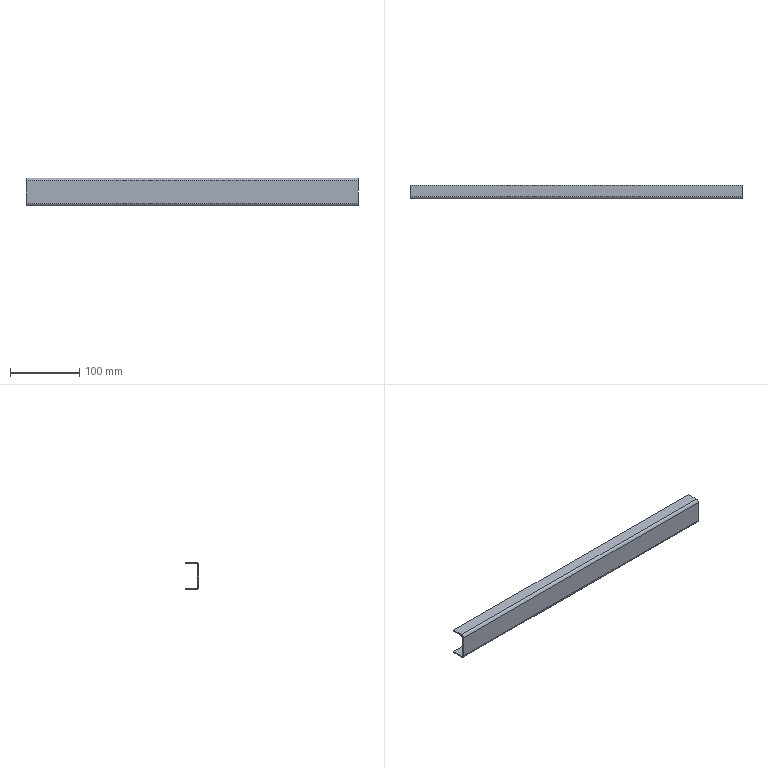Component | SolidWorks | ElectricalCabinetDoorAssembly-1_ElectricalCabinetDoorStiffener-1 | 1 solid | 22 faces | box 480 x 20 x 40 mm | volume 70488 mm3 | plane 18 | cylinder 4 | commonest cylinder face diameters 8 x2 4 x2 | material Plain Carbon Steel
STEP:
#1=COLOUR_RGB('',0.7922,0.8196,0.9333);
#2=FILL_AREA_STYLE_COLOUR('',#1);
#3=FILL_AREA_STYLE('',(#2));
#4=SURFACE_STYLE_FILL_AREA(#3);
#5=SURFACE_SIDE_STYLE('',(#4));
#6=SURFACE_STYLE_USAGE(.BOTH.,#5);
#7=PRESENTATION_STYLE_ASSIGNMENT((#6));
#8=CARTESIAN_POINT('',(96.921,48.88,54.212));
#9=VERTEX_POINT('',#8);
#10=CARTESIAN_POINT('',(96.921,48.959,54.212));
#11=VERTEX_POINT('',#10);
#12=CARTESIAN_POINT('',(96.921,48.88,54.212));
#13=DIRECTION('',(0.,1.,-0.));
#14=VECTOR('',#13,39.37);
#15=LINE('',#12,#14);
#16=EDGE_CURVE('',#9,#11,#15,.T.);
#17=ORIENTED_EDGE('',*,*,#16,.F.);
#18=CARTESIAN_POINT('',(96.921,49.037,54.054));
#19=VERTEX_POINT('',#18);
#20=CARTESIAN_POINT('',(96.921,49.037,54.212));
#21=DIRECTION('',(-1.,0.,0.));
#22=DIRECTION('',(0.,0.,1.));
#23=AXIS2_PLACEMENT_3D('',#20,#21,#22);
#24=CIRCLE('',#23,0.1575);
#25=EDGE_CURVE('',#19,#9,#24,.T.);
#26=ORIENTED_EDGE('',*,*,#25,.F.);
#27=CARTESIAN_POINT('',(96.921,49.037,54.133));
#28=VERTEX_POINT('',#27);
#29=CARTESIAN_POINT('',(96.921,49.037,54.133));
#30=DIRECTION('',(-0.,-0.,-1.));
#31=VECTOR('',#30,39.37);
#32=LINE('',#29,#31);
#33=EDGE_CURVE('',#28,#19,#32,.T.);
#34=ORIENTED_EDGE('',*,*,#33,.F.);
#35=CARTESIAN_POINT('',(96.921,49.037,54.212));
#36=DIRECTION('',(-1.,0.,0.));
#37=DIRECTION('',(0.,0.,1.));
#38=AXIS2_PLACEMENT_3D('',#35,#36,#37);
#39=CIRCLE('',#38,0.07874);
#40=EDGE_CURVE('',#28,#11,#39,.T.);
#41=ORIENTED_EDGE('',*,*,#40,.T.);
#42=EDGE_LOOP('',(#17,#26,#34,#41));
#43=FACE_OUTER_BOUND('',#42,.T.);
#44=CARTESIAN_POINT('',(96.921,48.88,54.212));
#45=DIRECTION('',(1.,-0.,-0.));
#46=DIRECTION('',(0.,0.,1.));
#47=AXIS2_PLACEMENT_3D('',#44,#45,#46);
#48=PLANE('',#47);
#49=ADVANCED_FACE('',(#43),#48,.T.);
#50=CARTESIAN_POINT('',(96.921,48.88,55.472));
#51=VERTEX_POINT('',#50);
#52=CARTESIAN_POINT('',(96.921,48.88,54.054));
#53=DIRECTION('',(0.,0.,1.));
#54=VECTOR('',#53,39.37);
#55=LINE('',#52,#54);
#56=EDGE_CURVE('',#9,#51,#55,.T.);
#57=ORIENTED_EDGE('',*,*,#56,.F.);
#58=ORIENTED_EDGE('',*,*,#16,.T.);
#59=CARTESIAN_POINT('',(96.921,48.959,55.472));
#60=VERTEX_POINT('',#59);
#61=CARTESIAN_POINT('',(96.921,48.959,54.054));
#62=DIRECTION('',(0.,0.,1.));
#63=VECTOR('',#62,39.37);
#64=LINE('',#61,#63);
#65=EDGE_CURVE('',#11,#60,#64,.T.);
#66=ORIENTED_EDGE('',*,*,#65,.T.);
#67=CARTESIAN_POINT('',(96.921,48.959,55.472));
#68=DIRECTION('',(-0.,-1.,0.));
#69=VECTOR('',#68,39.37);
#70=LINE('',#67,#69);
#71=EDGE_CURVE('',#60,#51,#70,.T.);
#72=ORIENTED_EDGE('',*,*,#71,.T.);
#73=EDGE_LOOP('',(#57,#58,#66,#72));
#74=FACE_OUTER_BOUND('',#73,.T.);
#75=CARTESIAN_POINT('',(96.921,49.037,54.133));
#76=DIRECTION('',(1.,-0.,-0.));
#77=DIRECTION('',(0.,0.,1.));
#78=AXIS2_PLACEMENT_3D('',#75,#76,#77);
#79=PLANE('',#78);
#80=ADVANCED_FACE('',(#74),#79,.T.);
#81=CARTESIAN_POINT('',(78.023,49.037,54.054));
#82=VERTEX_POINT('',#81);
#83=CARTESIAN_POINT('',(78.023,49.037,54.133));
#84=VERTEX_POINT('',#83);
#85=CARTESIAN_POINT('',(78.023,49.037,54.054));
#86=DIRECTION('',(0.,0.,1.));
#87=VECTOR('',#86,39.37);
#88=LINE('',#85,#87);
#89=EDGE_CURVE('',#82,#84,#88,.T.);
#90=ORIENTED_EDGE('',*,*,#89,.F.);
#91=CARTESIAN_POINT('',(78.023,48.88,54.212));
#92=VERTEX_POINT('',#91);
#93=CARTESIAN_POINT('',(78.023,49.037,54.212));
#94=DIRECTION('',(-1.,0.,0.));
#95=DIRECTION('',(0.,0.,1.));
#96=AXIS2_PLACEMENT_3D('',#93,#94,#95);
#97=CIRCLE('',#96,0.1575);
#98=EDGE_CURVE('',#82,#92,#97,.T.);
#99=ORIENTED_EDGE('',*,*,#98,.T.);
#100=CARTESIAN_POINT('',(78.023,48.959,54.212));
#101=VERTEX_POINT('',#100);
#102=CARTESIAN_POINT('',(78.023,48.959,54.212));
#103=DIRECTION('',(-0.,-1.,0.));
#104=VECTOR('',#103,39.37);
#105=LINE('',#102,#104);
#106=EDGE_CURVE('',#101,#92,#105,.T.);
#107=ORIENTED_EDGE('',*,*,#106,.F.);
#108=CARTESIAN_POINT('',(78.023,49.037,54.212));
#109=DIRECTION('',(-1.,0.,0.));
#110=DIRECTION('',(0.,0.,1.));
#111=AXIS2_PLACEMENT_3D('',#108,#109,#110);
#112=CIRCLE('',#111,0.07874);
#113=EDGE_CURVE('',#84,#101,#112,.T.);
#114=ORIENTED_EDGE('',*,*,#113,.F.);
#115=EDGE_LOOP('',(#90,#99,#107,#114));
#116=FACE_OUTER_BOUND('',#115,.T.);
#117=CARTESIAN_POINT('',(78.023,49.037,54.054));
#118=DIRECTION('',(-1.,0.,0.));
#119=DIRECTION('',(-0.,-0.,-1.));
#120=AXIS2_PLACEMENT_3D('',#117,#118,#119);
#121=PLANE('',#120);
#122=ADVANCED_FACE('',(#116),#121,.T.);
#123=CARTESIAN_POINT('',(78.023,49.667,54.054));
#124=VERTEX_POINT('',#123);
#125=CARTESIAN_POINT('',(78.023,49.667,54.054));
#126=DIRECTION('',(-0.,-1.,0.));
#127=VECTOR('',#126,39.37);
#128=LINE('',#125,#127);
#129=EDGE_CURVE('',#124,#82,#128,.T.);
#130=ORIENTED_EDGE('',*,*,#129,.T.);
#131=ORIENTED_EDGE('',*,*,#89,.T.);
#132=CARTESIAN_POINT('',(78.023,49.667,54.133));
#133=VERTEX_POINT('',#132);
#134=CARTESIAN_POINT('',(78.023,49.667,54.133));
#135=DIRECTION('',(-0.,-1.,0.));
#136=VECTOR('',#135,39.37);
#137=LINE('',#134,#136);
#138=EDGE_CURVE('',#133,#84,#137,.T.);
#139=ORIENTED_EDGE('',*,*,#138,.F.);
#140=CARTESIAN_POINT('',(78.023,49.667,54.133));
#141=DIRECTION('',(-0.,-0.,-1.));
#142=VECTOR('',#141,39.37);
#143=LINE('',#140,#142);
#144=EDGE_CURVE('',#133,#124,#143,.T.);
#145=ORIENTED_EDGE('',*,*,#144,.T.);
#146=EDGE_LOOP('',(#130,#131,#139,#145));
#147=FACE_OUTER_BOUND('',#146,.T.);
#148=CARTESIAN_POINT('',(78.023,48.959,54.212));
#149=DIRECTION('',(-1.,0.,0.));
#150=DIRECTION('',(-0.,-0.,-1.));
#151=AXIS2_PLACEMENT_3D('',#148,#149,#150);
#152=PLANE('',#151);
#153=ADVANCED_FACE('',(#147),#152,.T.);
#154=CARTESIAN_POINT('',(96.921,49.037,55.629));
#155=VERTEX_POINT('',#154);
#156=CARTESIAN_POINT('',(96.921,49.037,55.55));
#157=VERTEX_POINT('',#156);
#158=CARTESIAN_POINT('',(96.921,49.037,55.629));
#159=DIRECTION('',(-0.,-0.,-1.));
#160=VECTOR('',#159,39.37);
#161=LINE('',#158,#160);
#162=EDGE_CURVE('',#155,#157,#161,.T.);
#163=ORIENTED_EDGE('',*,*,#162,.F.);
#164=CARTESIAN_POINT('',(96.921,49.037,55.472));
#165=DIRECTION('',(-1.,0.,0.));
#166=DIRECTION('',(0.,0.,1.));
#167=AXIS2_PLACEMENT_3D('',#164,#165,#166);
#168=CIRCLE('',#167,0.1575);
#169=EDGE_CURVE('',#51,#155,#168,.T.);
#170=ORIENTED_EDGE('',*,*,#169,.F.);
#171=ORIENTED_EDGE('',*,*,#71,.F.);
#172=CARTESIAN_POINT('',(96.921,49.037,55.472));
#173=DIRECTION('',(-1.,0.,0.));
#174=DIRECTION('',(0.,0.,1.));
#175=AXIS2_PLACEMENT_3D('',#172,#173,#174);
#176=CIRCLE('',#175,0.07874);
#177=EDGE_CURVE('',#60,#157,#176,.T.);
#178=ORIENTED_EDGE('',*,*,#177,.T.);
#179=EDGE_LOOP('',(#163,#170,#171,#178));
#180=FACE_OUTER_BOUND('',#179,.T.);
#181=CARTESIAN_POINT('',(96.921,49.037,55.629));
#182=DIRECTION('',(1.,-0.,-0.));
#183=DIRECTION('',(0.,0.,1.));
#184=AXIS2_PLACEMENT_3D('',#181,#182,#183);
#185=PLANE('',#184);
#186=ADVANCED_FACE('',(#180),#185,.T.);
#187=CARTESIAN_POINT('',(96.921,49.667,55.629));
#188=VERTEX_POINT('',#187);
#189=CARTESIAN_POINT('',(96.921,48.88,55.629));
#190=DIRECTION('',(0.,1.,-0.));
#191=VECTOR('',#190,39.37);
#192=LINE('',#189,#191);
#193=EDGE_CURVE('',#155,#188,#192,.T.);
#194=ORIENTED_EDGE('',*,*,#193,.F.);
#195=ORIENTED_EDGE('',*,*,#162,.T.);
#196=CARTESIAN_POINT('',(96.921,49.667,55.55));
#197=VERTEX_POINT('',#196);
#198=CARTESIAN_POINT('',(96.921,48.88,55.55));
#199=DIRECTION('',(0.,1.,-0.));
#200=VECTOR('',#199,39.37);
#201=LINE('',#198,#200);
#202=EDGE_CURVE('',#157,#197,#201,.T.);
#203=ORIENTED_EDGE('',*,*,#202,.T.);
#204=CARTESIAN_POINT('',(96.921,49.667,55.629));
#205=DIRECTION('',(-0.,-0.,-1.));
#206=VECTOR('',#205,39.37);
#207=LINE('',#204,#206);
#208=EDGE_CURVE('',#188,#197,#207,.T.);
#209=ORIENTED_EDGE('',*,*,#208,.F.);
#210=EDGE_LOOP('',(#194,#195,#203,#209));
#211=FACE_OUTER_BOUND('',#210,.T.);
#212=CARTESIAN_POINT('',(96.921,48.959,55.472));
#213=DIRECTION('',(1.,-0.,-0.));
#214=DIRECTION('',(0.,0.,1.));
#215=AXIS2_PLACEMENT_3D('',#212,#213,#214);
#216=PLANE('',#215);
#217=ADVANCED_FACE('',(#211),#216,.T.);
#218=CARTESIAN_POINT('',(78.023,48.88,55.472));
#219=VERTEX_POINT('',#218);
#220=CARTESIAN_POINT('',(78.023,48.959,55.472));
#221=VERTEX_POINT('',#220);
#222=CARTESIAN_POINT('',(78.023,48.88,55.472));
#223=DIRECTION('',(0.,1.,-0.));
#224=VECTOR('',#223,39.37);
#225=LINE('',#222,#224);
#226=EDGE_CURVE('',#219,#221,#225,.T.);
#227=ORIENTED_EDGE('',*,*,#226,.F.);
#228=CARTESIAN_POINT('',(78.023,49.037,55.629));
#229=VERTEX_POINT('',#228);
#230=CARTESIAN_POINT('',(78.023,49.037,55.472));
#231=DIRECTION('',(-1.,0.,0.));
#232=DIRECTION('',(0.,0.,1.));
#233=AXIS2_PLACEMENT_3D('',#230,#231,#232);
#234=CIRCLE('',#233,0.1575);
#235=EDGE_CURVE('',#219,#229,#234,.T.);
#236=ORIENTED_EDGE('',*,*,#235,.T.);
#237=CARTESIAN_POINT('',(78.023,49.037,55.55));
#238=VERTEX_POINT('',#237);
#239=CARTESIAN_POINT('',(78.023,49.037,55.55));
#240=DIRECTION('',(0.,0.,1.));
#241=VECTOR('',#240,39.37);
#242=LINE('',#239,#241);
#243=EDGE_CURVE('',#238,#229,#242,.T.);
#244=ORIENTED_EDGE('',*,*,#243,.F.);
#245=CARTESIAN_POINT('',(78.023,49.037,55.472));
#246=DIRECTION('',(-1.,0.,0.));
#247=DIRECTION('',(0.,0.,1.));
#248=AXIS2_PLACEMENT_3D('',#245,#246,#247);
#249=CIRCLE('',#248,0.07874);
#250=EDGE_CURVE('',#221,#238,#249,.T.);
#251=ORIENTED_EDGE('',*,*,#250,.F.);
#252=EDGE_LOOP('',(#227,#236,#244,#251));
#253=FACE_OUTER_BOUND('',#252,.T.);
#254=CARTESIAN_POINT('',(78.023,48.88,55.472));
#255=DIRECTION('',(-1.,0.,0.));
#256=DIRECTION('',(-0.,-0.,-1.));
#257=AXIS2_PLACEMENT_3D('',#254,#255,#256);
#258=PLANE('',#257);
#259=ADVANCED_FACE('',(#253),#258,.T.);
#260=CARTESIAN_POINT('',(78.023,48.88,54.054));
#261=DIRECTION('',(0.,0.,1.));
#262=VECTOR('',#261,39.37);
#263=LINE('',#260,#262);
#264=EDGE_CURVE('',#92,#219,#263,.T.);
#265=ORIENTED_EDGE('',*,*,#264,.T.);
#266=ORIENTED_EDGE('',*,*,#226,.T.);
#267=CARTESIAN_POINT('',(78.023,48.959,54.054));
#268=DIRECTION('',(0.,0.,1.));
#269=VECTOR('',#268,39.37);
#270=LINE('',#267,#269);
#271=EDGE_CURVE('',#101,#221,#270,.T.);
#272=ORIENTED_EDGE('',*,*,#271,.F.);
#273=ORIENTED_EDGE('',*,*,#106,.T.);
#274=EDGE_LOOP('',(#265,#266,#272,#273));
#275=FACE_OUTER_BOUND('',#274,.T.);
#276=CARTESIAN_POINT('',(78.023,49.037,55.55));
#277=DIRECTION('',(-1.,0.,0.));
#278=DIRECTION('',(-0.,-0.,-1.));
#279=AXIS2_PLACEMENT_3D('',#276,#277,#278);
#280=PLANE('',#279);
#281=ADVANCED_FACE('',(#275),#280,.T.);
#282=CARTESIAN_POINT('',(78.023,49.667,55.55));
#283=VERTEX_POINT('',#282);
#284=CARTESIAN_POINT('',(78.023,48.88,55.55));
#285=DIRECTION('',(0.,1.,-0.));
#286=VECTOR('',#285,39.37);
#287=LINE('',#284,#286);
#288=EDGE_CURVE('',#238,#283,#287,.T.);
#289=ORIENTED_EDGE('',*,*,#288,.T.);
#290=CARTESIAN_POINT('',(96.921,49.667,55.55));
#291=DIRECTION('',(-1.,0.,0.));
#292=VECTOR('',#291,39.37);
#293=LINE('',#290,#292);
#294=EDGE_CURVE('',#197,#283,#293,.T.);
#295=ORIENTED_EDGE('',*,*,#294,.F.);
#296=ORIENTED_EDGE('',*,*,#202,.F.);
#297=CARTESIAN_POINT('',(96.921,49.037,55.55));
#298=DIRECTION('',(-1.,0.,0.));
#299=VECTOR('',#298,39.37);
#300=LINE('',#297,#299);
#301=EDGE_CURVE('',#157,#238,#300,.T.);
#302=ORIENTED_EDGE('',*,*,#301,.T.);
#303=EDGE_LOOP('',(#289,#295,#296,#302));
#304=FACE_OUTER_BOUND('',#303,.T.);
#305=CARTESIAN_POINT('',(96.921,48.88,55.55));
#306=DIRECTION('',(0.,0.,1.));
#307=DIRECTION('',(-1.,0.,0.));
#308=AXIS2_PLACEMENT_3D('',#305,#306,#307);
#309=PLANE('',#308);
#310=ADVANCED_FACE('',(#304),#309,.F.);
#311=CARTESIAN_POINT('',(78.023,49.667,55.629));
#312=VERTEX_POINT('',#311);
#313=CARTESIAN_POINT('',(78.023,49.667,55.629));
#314=DIRECTION('',(-0.,-0.,-1.));
#315=VECTOR('',#314,39.37);
#316=LINE('',#313,#315);
#317=EDGE_CURVE('',#312,#283,#316,.T.);
#318=ORIENTED_EDGE('',*,*,#317,.F.);
#319=CARTESIAN_POINT('',(96.921,49.667,55.629));
#320=DIRECTION('',(-1.,0.,0.));
#321=VECTOR('',#320,39.37);
#322=LINE('',#319,#321);
#323=EDGE_CURVE('',#188,#312,#322,.T.);
#324=ORIENTED_EDGE('',*,*,#323,.F.);
#325=ORIENTED_EDGE('',*,*,#208,.T.);
#326=ORIENTED_EDGE('',*,*,#294,.T.);
#327=EDGE_LOOP('',(#318,#324,#325,#326));
#328=FACE_OUTER_BOUND('',#327,.T.);
#329=CARTESIAN_POINT('',(96.921,49.667,55.629));
#330=DIRECTION('',(0.,1.,-0.));
#331=DIRECTION('',(-1.,0.,0.));
#332=AXIS2_PLACEMENT_3D('',#329,#330,#331);
#333=PLANE('',#332);
#334=ADVANCED_FACE('',(#328),#333,.T.);
#335=CARTESIAN_POINT('',(78.023,48.88,55.629));
#336=DIRECTION('',(0.,1.,-0.));
#337=VECTOR('',#336,39.37);
#338=LINE('',#335,#337);
#339=EDGE_CURVE('',#229,#312,#338,.T.);
#340=ORIENTED_EDGE('',*,*,#339,.F.);
#341=CARTESIAN_POINT('',(96.921,49.037,55.629));
#342=DIRECTION('',(-1.,0.,0.));
#343=VECTOR('',#342,39.37);
#344=LINE('',#341,#343);
#345=EDGE_CURVE('',#155,#229,#344,.T.);
#346=ORIENTED_EDGE('',*,*,#345,.F.);
#347=ORIENTED_EDGE('',*,*,#193,.T.);
#348=ORIENTED_EDGE('',*,*,#323,.T.);
#349=EDGE_LOOP('',(#340,#346,#347,#348));
#350=FACE_OUTER_BOUND('',#349,.T.);
#351=CARTESIAN_POINT('',(96.921,48.88,55.629));
#352=DIRECTION('',(0.,0.,1.));
#353=DIRECTION('',(-1.,0.,0.));
#354=AXIS2_PLACEMENT_3D('',#351,#352,#353);
#355=PLANE('',#354);
#356=ADVANCED_FACE('',(#350),#355,.T.);
#357=ORIENTED_EDGE('',*,*,#235,.F.);
#358=CARTESIAN_POINT('',(96.921,48.88,55.472));
#359=DIRECTION('',(-1.,0.,0.));
#360=VECTOR('',#359,39.37);
#361=LINE('',#358,#360);
#362=EDGE_CURVE('',#51,#219,#361,.T.);
#363=ORIENTED_EDGE('',*,*,#362,.F.);
#364=ORIENTED_EDGE('',*,*,#169,.T.);
#365=ORIENTED_EDGE('',*,*,#345,.T.);
#366=EDGE_LOOP('',(#357,#363,#364,#365));
#367=FACE_OUTER_BOUND('',#366,.T.);
#368=CARTESIAN_POINT('',(96.921,49.037,55.472));
#369=DIRECTION('',(-1.,0.,0.));
#370=DIRECTION('',(0.,0.,-1.));
#371=AXIS2_PLACEMENT_3D('',#368,#369,#370);
#372=CYLINDRICAL_SURFACE('',#371,0.1575);
#373=ADVANCED_FACE('',(#367),#372,.T.);
#374=ORIENTED_EDGE('',*,*,#264,.F.);
#375=CARTESIAN_POINT('',(96.921,48.88,54.212));
#376=DIRECTION('',(-1.,0.,0.));
#377=VECTOR('',#376,39.37);
#378=LINE('',#375,#377);
#379=EDGE_CURVE('',#9,#92,#378,.T.);
#380=ORIENTED_EDGE('',*,*,#379,.F.);
#381=ORIENTED_EDGE('',*,*,#56,.T.);
#382=ORIENTED_EDGE('',*,*,#362,.T.);
#383=EDGE_LOOP('',(#374,#380,#381,#382));
#384=FACE_OUTER_BOUND('',#383,.T.);
#385=CARTESIAN_POINT('',(96.921,48.88,54.054));
#386=DIRECTION('',(-0.,-1.,0.));
#387=DIRECTION('',(1.,-0.,-0.));
#388=AXIS2_PLACEMENT_3D('',#385,#386,#387);
#389=PLANE('',#388);
#390=ADVANCED_FACE('',(#384),#389,.T.);
#391=ORIENTED_EDGE('',*,*,#98,.F.);
#392=CARTESIAN_POINT('',(96.921,49.037,54.054));
#393=DIRECTION('',(-1.,0.,0.));
#394=VECTOR('',#393,39.37);
#395=LINE('',#392,#394);
#396=EDGE_CURVE('',#19,#82,#395,.T.);
#397=ORIENTED_EDGE('',*,*,#396,.F.);
#398=ORIENTED_EDGE('',*,*,#25,.T.);
#399=ORIENTED_EDGE('',*,*,#379,.T.);
#400=EDGE_LOOP('',(#391,#397,#398,#399));
#401=FACE_OUTER_BOUND('',#400,.T.);
#402=CARTESIAN_POINT('',(96.921,49.037,54.212));
#403=DIRECTION('',(-1.,0.,0.));
#404=DIRECTION('',(0.,0.,-1.));
#405=AXIS2_PLACEMENT_3D('',#402,#403,#404);
#406=CYLINDRICAL_SURFACE('',#405,0.1575);
#407=ADVANCED_FACE('',(#401),#406,.T.);
#408=ORIENTED_EDGE('',*,*,#129,.F.);
#409=CARTESIAN_POINT('',(96.921,49.667,54.054));
#410=VERTEX_POINT('',#409);
#411=CARTESIAN_POINT('',(96.921,49.667,54.054));
#412=DIRECTION('',(-1.,0.,0.));
#413=VECTOR('',#412,39.37);
#414=LINE('',#411,#413);
#415=EDGE_CURVE('',#410,#124,#414,.T.);
#416=ORIENTED_EDGE('',*,*,#415,.F.);
#417=CARTESIAN_POINT('',(96.921,49.667,54.054));
#418=DIRECTION('',(-0.,-1.,0.));
#419=VECTOR('',#418,39.37);
#420=LINE('',#417,#419);
#421=EDGE_CURVE('',#410,#19,#420,.T.);
#422=ORIENTED_EDGE('',*,*,#421,.T.);
#423=ORIENTED_EDGE('',*,*,#396,.T.);
#424=EDGE_LOOP('',(#408,#416,#422,#423));
#425=FACE_OUTER_BOUND('',#424,.T.);
#426=CARTESIAN_POINT('',(96.921,49.667,54.054));
#427=DIRECTION('',(-0.,-0.,-1.));
#428=DIRECTION('',(1.,-0.,-0.));
#429=AXIS2_PLACEMENT_3D('',#426,#427,#428);
#430=PLANE('',#429);
#431=ADVANCED_FACE('',(#425),#430,.T.);
#432=ORIENTED_EDGE('',*,*,#144,.F.);
#433=CARTESIAN_POINT('',(96.921,49.667,54.133));
#434=VERTEX_POINT('',#433);
#435=CARTESIAN_POINT('',(96.921,49.667,54.133));
#436=DIRECTION('',(-1.,0.,0.));
#437=VECTOR('',#436,39.37);
#438=LINE('',#435,#437);
#439=EDGE_CURVE('',#434,#133,#438,.T.);
#440=ORIENTED_EDGE('',*,*,#439,.F.);
#441=CARTESIAN_POINT('',(96.921,49.667,54.133));
#442=DIRECTION('',(-0.,-0.,-1.));
#443=VECTOR('',#442,39.37);
#444=LINE('',#441,#443);
#445=EDGE_CURVE('',#434,#410,#444,.T.);
#446=ORIENTED_EDGE('',*,*,#445,.T.);
#447=ORIENTED_EDGE('',*,*,#415,.T.);
#448=EDGE_LOOP('',(#432,#440,#446,#447));
#449=FACE_OUTER_BOUND('',#448,.T.);
#450=CARTESIAN_POINT('',(96.921,49.667,54.133));
#451=DIRECTION('',(0.,1.,-0.));
#452=DIRECTION('',(-1.,0.,0.));
#453=AXIS2_PLACEMENT_3D('',#450,#451,#452);
#454=PLANE('',#453);
#455=ADVANCED_FACE('',(#449),#454,.T.);
#456=ORIENTED_EDGE('',*,*,#138,.T.);
#457=CARTESIAN_POINT('',(96.921,49.037,54.133));
#458=DIRECTION('',(-1.,0.,0.));
#459=VECTOR('',#458,39.37);
#460=LINE('',#457,#459);
#461=EDGE_CURVE('',#28,#84,#460,.T.);
#462=ORIENTED_EDGE('',*,*,#461,.F.);
#463=CARTESIAN_POINT('',(96.921,49.667,54.133));
#464=DIRECTION('',(-0.,-1.,0.));
#465=VECTOR('',#464,39.37);
#466=LINE('',#463,#465);
#467=EDGE_CURVE('',#434,#28,#466,.T.);
#468=ORIENTED_EDGE('',*,*,#467,.F.);
#469=ORIENTED_EDGE('',*,*,#439,.T.);
#470=EDGE_LOOP('',(#456,#462,#468,#469));
#471=FACE_OUTER_BOUND('',#470,.T.);
#472=CARTESIAN_POINT('',(96.921,49.667,54.133));
#473=DIRECTION('',(-0.,-0.,-1.));
#474=DIRECTION('',(1.,-0.,-0.));
#475=AXIS2_PLACEMENT_3D('',#472,#473,#474);
#476=PLANE('',#475);
#477=ADVANCED_FACE('',(#471),#476,.F.);
#478=ORIENTED_EDGE('',*,*,#113,.T.);
#479=CARTESIAN_POINT('',(96.921,48.959,54.212));
#480=DIRECTION('',(-1.,0.,0.));
#481=VECTOR('',#480,39.37);
#482=LINE('',#479,#481);
#483=EDGE_CURVE('',#11,#101,#482,.T.);
#484=ORIENTED_EDGE('',*,*,#483,.F.);
#485=ORIENTED_EDGE('',*,*,#40,.F.);
#486=ORIENTED_EDGE('',*,*,#461,.T.);
#487=EDGE_LOOP('',(#478,#484,#485,#486));
#488=FACE_OUTER_BOUND('',#487,.T.);
#489=CARTESIAN_POINT('',(96.921,49.037,54.212));
#490=DIRECTION('',(-1.,0.,0.));
#491=DIRECTION('',(0.,0.,-1.));
#492=AXIS2_PLACEMENT_3D('',#489,#490,#491);
#493=CYLINDRICAL_SURFACE('',#492,0.07874);
#494=ADVANCED_FACE('',(#488),#493,.F.);
#495=ORIENTED_EDGE('',*,*,#271,.T.);
#496=CARTESIAN_POINT('',(96.921,48.959,55.472));
#497=DIRECTION('',(-1.,0.,0.));
#498=VECTOR('',#497,39.37);
#499=LINE('',#496,#498);
#500=EDGE_CURVE('',#60,#221,#499,.T.);
#501=ORIENTED_EDGE('',*,*,#500,.F.);
#502=ORIENTED_EDGE('',*,*,#65,.F.);
#503=ORIENTED_EDGE('',*,*,#483,.T.);
#504=EDGE_LOOP('',(#495,#501,#502,#503));
#505=FACE_OUTER_BOUND('',#504,.T.);
#506=CARTESIAN_POINT('',(96.921,48.959,54.054));
#507=DIRECTION('',(-0.,-1.,0.));
#508=DIRECTION('',(1.,-0.,-0.));
#509=AXIS2_PLACEMENT_3D('',#506,#507,#508);
#510=PLANE('',#509);
#511=ADVANCED_FACE('',(#505),#510,.F.);
#512=ORIENTED_EDGE('',*,*,#250,.T.);
#513=ORIENTED_EDGE('',*,*,#301,.F.);
#514=ORIENTED_EDGE('',*,*,#177,.F.);
#515=ORIENTED_EDGE('',*,*,#500,.T.);
#516=EDGE_LOOP('',(#512,#513,#514,#515));
#517=FACE_OUTER_BOUND('',#516,.T.);
#518=CARTESIAN_POINT('',(96.921,49.037,55.472));
#519=DIRECTION('',(-1.,0.,0.));
#520=DIRECTION('',(0.,0.,-1.));
#521=AXIS2_PLACEMENT_3D('',#518,#519,#520);
#522=CYLINDRICAL_SURFACE('',#521,0.07874);
#523=ADVANCED_FACE('',(#517),#522,.F.);
#524=ORIENTED_EDGE('',*,*,#467,.T.);
#525=ORIENTED_EDGE('',*,*,#33,.T.);
#526=ORIENTED_EDGE('',*,*,#421,.F.);
#527=ORIENTED_EDGE('',*,*,#445,.F.);
#528=EDGE_LOOP('',(#524,#525,#526,#527));
#529=FACE_OUTER_BOUND('',#528,.T.);
#530=CARTESIAN_POINT('',(96.921,49.037,55.472));
#531=DIRECTION('',(1.,-0.,-0.));
#532=DIRECTION('',(0.,0.,1.));
#533=AXIS2_PLACEMENT_3D('',#530,#531,#532);
#534=PLANE('',#533);
#535=ADVANCED_FACE('',(#529),#534,.T.);
#536=ORIENTED_EDGE('',*,*,#288,.F.);
#537=ORIENTED_EDGE('',*,*,#243,.T.);
#538=ORIENTED_EDGE('',*,*,#339,.T.);
#539=ORIENTED_EDGE('',*,*,#317,.T.);
#540=EDGE_LOOP('',(#536,#537,#538,#539));
#541=FACE_OUTER_BOUND('',#540,.T.);
#542=CARTESIAN_POINT('',(78.023,49.037,55.472));
#543=DIRECTION('',(1.,-0.,-0.));
#544=DIRECTION('',(0.,0.,1.));
#545=AXIS2_PLACEMENT_3D('',#542,#543,#544);
#546=PLANE('',#545);
#547=ADVANCED_FACE('',(#541),#546,.F.);
#548=CLOSED_SHELL('',(#49,#80,#122,#153,#186,#217,#259,#281,#310,#334,#356,#373,#390,#407,#431,#455,#477,#494,#511,#523,#535,#547));
#549=MANIFOLD_SOLID_BREP('',#548);
#550=STYLED_ITEM('',(#7),#549);
#551=PRESENTATION_LAYER_ASSIGNMENT('','',(#550));
#552=(LENGTH_UNIT()NAMED_UNIT(*)SI_UNIT($,.METRE.));
#553=LENGTH_MEASURE_WITH_UNIT(LENGTH_MEASURE(0.0254),#552);
#554=DIMENSIONAL_EXPONENTS(1.,0.,0.,0.,0.,0.,0.);
#555=(CONVERSION_BASED_UNIT('',#553)LENGTH_UNIT()NAMED_UNIT(#554));
#556=UNCERTAINTY_MEASURE_WITH_UNIT(LENGTH_MEASURE(0.00001),#555,'','');
#557=(NAMED_UNIT(*)PLANE_ANGLE_UNIT()SI_UNIT($,.RADIAN.));
#558=(NAMED_UNIT(*)SI_UNIT($,.STERADIAN.)SOLID_ANGLE_UNIT());
#559=(GEOMETRIC_REPRESENTATION_CONTEXT(3)GLOBAL_UNCERTAINTY_ASSIGNED_CONTEXT((#556))GLOBAL_UNIT_ASSIGNED_CONTEXT((#555,#557,#558))REPRESENTATION_CONTEXT('',''));
#560=MECHANICAL_DESIGN_GEOMETRIC_PRESENTATION_REPRESENTATION('',(#550),#559);
#561=CARTESIAN_POINT('',(0.,0.,0.));
#562=DIRECTION('',(0.,0.,1.));
#563=DIRECTION('',(1.,0.,0.));
#564=AXIS2_PLACEMENT_3D('',#561,#562,#563);
#565=(LENGTH_UNIT()NAMED_UNIT(*)SI_UNIT($,.METRE.));
#566=LENGTH_MEASURE_WITH_UNIT(LENGTH_MEASURE(0.0254),#565);
#567=DIMENSIONAL_EXPONENTS(1.,0.,0.,0.,0.,0.,0.);
#568=(CONVERSION_BASED_UNIT('',#566)LENGTH_UNIT()NAMED_UNIT(#567));
#569=UNCERTAINTY_MEASURE_WITH_UNIT(LENGTH_MEASURE(0.00001),#568,'','');
#570=(NAMED_UNIT(*)PLANE_ANGLE_UNIT()SI_UNIT($,.RADIAN.));
#571=(NAMED_UNIT(*)SI_UNIT($,.STERADIAN.)SOLID_ANGLE_UNIT());
#572=(GEOMETRIC_REPRESENTATION_CONTEXT(3)GLOBAL_UNCERTAINTY_ASSIGNED_CONTEXT((#569))GLOBAL_UNIT_ASSIGNED_CONTEXT((#568,#570,#571))REPRESENTATION_CONTEXT('',''));
#573=ADVANCED_BREP_SHAPE_REPRESENTATION('',(#549,#564),#572);